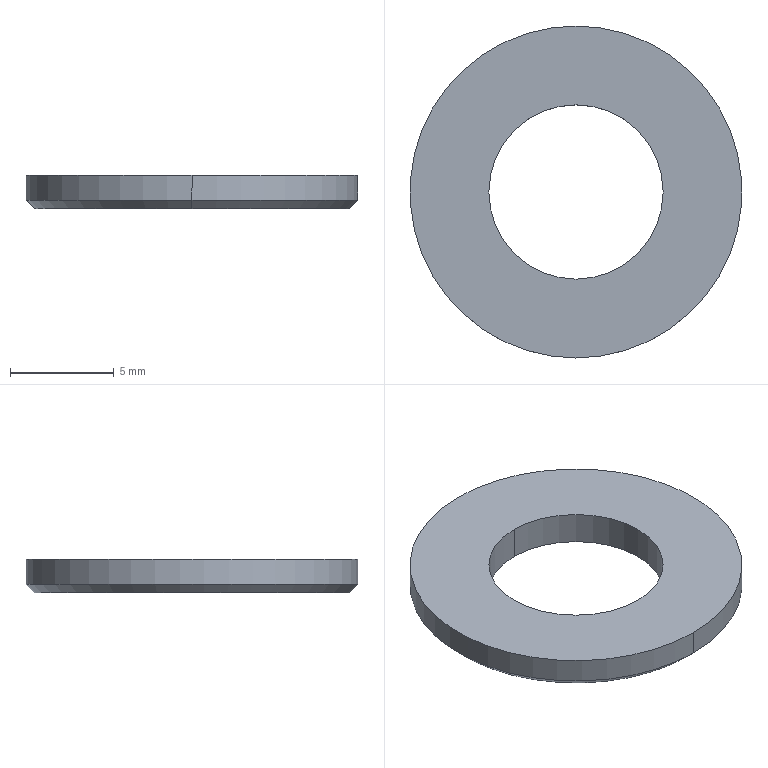Component | SolidWorks | GB_T97.2-1985FlatWasherChamferedTypeA8x1.6-10 | 1 solid | 8 faces | box 16 x 16 x 1.6 mm | volume 229 mm3 | cylinder 4 | cone 2 | plane 2 | commonest cylinder face diameters 16 x2 8.4 x2 | material Steel
build123d program:
from build123d import *


with BuildPart() as part:
    # Sketch1 → Base-Revolve (revolve)
    with BuildSketch(Plane.XY, mode=Mode.PRIVATE) as base_revolve_sk:
        Polygon((-7.6, 10.245), (-8, 9.845), (-8, 8.645), (-4.2, 8.645), (-4.2, 10.245), align=None)
    revolve(base_revolve_sk.sketch.rotate(Axis((0, 0, 0), (0, 1, 0)), 270), axis=Axis((0, 0, 0), (0, 1, 0)))


solid = part.part

# Placed as in the assembly
solid = solid.moved(Location((280, -19, -26.355), (-90, 0, 0)))
STEP:
#1=CARTESIAN_POINT('',(11.024,-1.063,-1.425));
#2=VERTEX_POINT('',#1);
#3=CARTESIAN_POINT('',(11.024,-0.4331,-1.425));
#4=VERTEX_POINT('',#3);
#5=CARTESIAN_POINT('',(11.024,-0.748,-1.425));
#6=DIRECTION('',(-0.,-0.,1.));
#7=DIRECTION('',(0.,-1.,-0.));
#8=AXIS2_PLACEMENT_3D('',#5,#6,#7);
#9=CIRCLE('',#8,0.315);
#10=EDGE_CURVE('',#2,#4,#9,.T.);
#11=ORIENTED_EDGE('',*,*,#10,.T.);
#12=CARTESIAN_POINT('',(11.024,-0.4331,-1.378));
#13=VERTEX_POINT('',#12);
#14=CARTESIAN_POINT('',(11.024,-0.4331,-1.038));
#15=DIRECTION('',(-0.,-0.,1.));
#16=VECTOR('',#15,39.37);
#17=LINE('',#14,#16);
#18=EDGE_CURVE('',#4,#13,#17,.T.);
#19=ORIENTED_EDGE('',*,*,#18,.T.);
#20=CARTESIAN_POINT('',(11.024,-1.063,-1.378));
#21=VERTEX_POINT('',#20);
#22=CARTESIAN_POINT('',(11.024,-0.748,-1.378));
#23=DIRECTION('',(-0.,-0.,1.));
#24=DIRECTION('',(0.,-1.,-0.));
#25=AXIS2_PLACEMENT_3D('',#22,#23,#24);
#26=CIRCLE('',#25,0.315);
#27=EDGE_CURVE('',#21,#13,#26,.T.);
#28=ORIENTED_EDGE('',*,*,#27,.F.);
#29=CARTESIAN_POINT('',(11.024,-1.063,-1.038));
#30=DIRECTION('',(-0.,-0.,1.));
#31=VECTOR('',#30,39.37);
#32=LINE('',#29,#31);
#33=EDGE_CURVE('',#2,#21,#32,.T.);
#34=ORIENTED_EDGE('',*,*,#33,.F.);
#35=EDGE_LOOP('',(#11,#19,#28,#34));
#36=FACE_OUTER_BOUND('',#35,.T.);
#37=CARTESIAN_POINT('',(11.024,-0.748,-1.038));
#38=DIRECTION('',(-0.,-0.,1.));
#39=DIRECTION('',(0.,-1.,-0.));
#40=AXIS2_PLACEMENT_3D('',#37,#38,#39);
#41=CYLINDRICAL_SURFACE('',#40,0.315);
#42=ADVANCED_FACE('',(#36),#41,.T.);
#43=CARTESIAN_POINT('',(11.024,-1.047,-1.441));
#44=VERTEX_POINT('',#43);
#45=CARTESIAN_POINT('',(11.024,-0.4488,-1.441));
#46=VERTEX_POINT('',#45);
#47=CARTESIAN_POINT('',(11.024,-0.748,-1.441));
#48=DIRECTION('',(-0.,-0.,1.));
#49=DIRECTION('',(0.,-1.,-0.));
#50=AXIS2_PLACEMENT_3D('',#47,#48,#49);
#51=CIRCLE('',#50,0.2992);
#52=EDGE_CURVE('',#44,#46,#51,.T.);
#53=ORIENTED_EDGE('',*,*,#52,.T.);
#54=CARTESIAN_POINT('',(11.024,-0.4488,-1.441));
#55=DIRECTION('',(-0.,0.7071,0.7071));
#56=VECTOR('',#55,39.37);
#57=LINE('',#54,#56);
#58=EDGE_CURVE('',#46,#4,#57,.T.);
#59=ORIENTED_EDGE('',*,*,#58,.T.);
#60=ORIENTED_EDGE('',*,*,#10,.F.);
#61=CARTESIAN_POINT('',(11.024,-1.047,-1.441));
#62=DIRECTION('',(-0.,-0.7071,0.7071));
#63=VECTOR('',#62,39.37);
#64=LINE('',#61,#63);
#65=EDGE_CURVE('',#44,#2,#64,.T.);
#66=ORIENTED_EDGE('',*,*,#65,.F.);
#67=EDGE_LOOP('',(#53,#59,#60,#66));
#68=FACE_OUTER_BOUND('',#67,.T.);
#69=CARTESIAN_POINT('',(11.024,-0.748,-1.441));
#70=DIRECTION('',(-0.,-0.,1.));
#71=DIRECTION('',(0.,-1.,-0.));
#72=AXIS2_PLACEMENT_3D('',#69,#70,#71);
#73=CONICAL_SURFACE('',#72,0.2992,0.7854);
#74=ADVANCED_FACE('',(#68),#73,.T.);
#75=CARTESIAN_POINT('',(11.024,-0.5827,-1.441));
#76=VERTEX_POINT('',#75);
#77=CARTESIAN_POINT('',(11.024,-0.9134,-1.441));
#78=VERTEX_POINT('',#77);
#79=CARTESIAN_POINT('',(11.024,-0.748,-1.441));
#80=DIRECTION('',(-0.,-0.,1.));
#81=DIRECTION('',(0.,-1.,-0.));
#82=AXIS2_PLACEMENT_3D('',#79,#80,#81);
#83=CIRCLE('',#82,0.1654);
#84=EDGE_CURVE('',#76,#78,#83,.T.);
#85=ORIENTED_EDGE('',*,*,#84,.F.);
#86=CARTESIAN_POINT('',(11.024,-0.5827,-1.378));
#87=VERTEX_POINT('',#86);
#88=CARTESIAN_POINT('',(11.024,-0.5827,-1.038));
#89=DIRECTION('',(-0.,-0.,1.));
#90=VECTOR('',#89,39.37);
#91=LINE('',#88,#90);
#92=EDGE_CURVE('',#76,#87,#91,.T.);
#93=ORIENTED_EDGE('',*,*,#92,.T.);
#94=CARTESIAN_POINT('',(11.024,-0.9134,-1.378));
#95=VERTEX_POINT('',#94);
#96=CARTESIAN_POINT('',(11.024,-0.748,-1.378));
#97=DIRECTION('',(-0.,-0.,1.));
#98=DIRECTION('',(0.,-1.,-0.));
#99=AXIS2_PLACEMENT_3D('',#96,#97,#98);
#100=CIRCLE('',#99,0.1654);
#101=EDGE_CURVE('',#87,#95,#100,.T.);
#102=ORIENTED_EDGE('',*,*,#101,.T.);
#103=CARTESIAN_POINT('',(11.024,-0.9134,-1.038));
#104=DIRECTION('',(-0.,-0.,1.));
#105=VECTOR('',#104,39.37);
#106=LINE('',#103,#105);
#107=EDGE_CURVE('',#78,#95,#106,.T.);
#108=ORIENTED_EDGE('',*,*,#107,.F.);
#109=EDGE_LOOP('',(#85,#93,#102,#108));
#110=FACE_OUTER_BOUND('',#109,.T.);
#111=CARTESIAN_POINT('',(11.024,-0.748,-1.038));
#112=DIRECTION('',(-0.,-0.,1.));
#113=DIRECTION('',(0.,-1.,-0.));
#114=AXIS2_PLACEMENT_3D('',#111,#112,#113);
#115=CYLINDRICAL_SURFACE('',#114,0.1654);
#116=ADVANCED_FACE('',(#110),#115,.F.);
#117=ORIENTED_EDGE('',*,*,#92,.F.);
#118=CARTESIAN_POINT('',(11.024,-0.748,-1.441));
#119=DIRECTION('',(-0.,-0.,1.));
#120=DIRECTION('',(0.,-1.,-0.));
#121=AXIS2_PLACEMENT_3D('',#118,#119,#120);
#122=CIRCLE('',#121,0.1654);
#123=EDGE_CURVE('',#78,#76,#122,.T.);
#124=ORIENTED_EDGE('',*,*,#123,.F.);
#125=ORIENTED_EDGE('',*,*,#107,.T.);
#126=CARTESIAN_POINT('',(11.024,-0.748,-1.378));
#127=DIRECTION('',(-0.,-0.,1.));
#128=DIRECTION('',(0.,-1.,-0.));
#129=AXIS2_PLACEMENT_3D('',#126,#127,#128);
#130=CIRCLE('',#129,0.1654);
#131=EDGE_CURVE('',#95,#87,#130,.T.);
#132=ORIENTED_EDGE('',*,*,#131,.T.);
#133=EDGE_LOOP('',(#117,#124,#125,#132));
#134=FACE_OUTER_BOUND('',#133,.T.);
#135=CARTESIAN_POINT('',(11.024,-0.748,-1.038));
#136=DIRECTION('',(-0.,-0.,1.));
#137=DIRECTION('',(0.,-1.,-0.));
#138=AXIS2_PLACEMENT_3D('',#135,#136,#137);
#139=CYLINDRICAL_SURFACE('',#138,0.1654);
#140=ADVANCED_FACE('',(#134),#139,.F.);
#141=ORIENTED_EDGE('',*,*,#52,.F.);
#142=CARTESIAN_POINT('',(11.024,-0.748,-1.441));
#143=DIRECTION('',(-0.,-0.,1.));
#144=DIRECTION('',(0.,-1.,-0.));
#145=AXIS2_PLACEMENT_3D('',#142,#143,#144);
#146=CIRCLE('',#145,0.2992);
#147=EDGE_CURVE('',#46,#44,#146,.T.);
#148=ORIENTED_EDGE('',*,*,#147,.F.);
#149=EDGE_LOOP('',(#141,#148));
#150=FACE_OUTER_BOUND('',#149,.T.);
#151=ORIENTED_EDGE('',*,*,#123,.T.);
#152=ORIENTED_EDGE('',*,*,#84,.T.);
#153=EDGE_LOOP('',(#151,#152));
#154=FACE_BOUND('',#153,.T.);
#155=CARTESIAN_POINT('',(10.858,-0.748,-1.441));
#156=DIRECTION('',(-0.,-0.,1.));
#157=DIRECTION('',(0.,-1.,-0.));
#158=AXIS2_PLACEMENT_3D('',#155,#156,#157);
#159=PLANE('',#158);
#160=ADVANCED_FACE('',(#150,#154),#159,.F.);
#161=ORIENTED_EDGE('',*,*,#58,.F.);
#162=ORIENTED_EDGE('',*,*,#147,.T.);
#163=ORIENTED_EDGE('',*,*,#65,.T.);
#164=CARTESIAN_POINT('',(11.024,-0.748,-1.425));
#165=DIRECTION('',(-0.,-0.,1.));
#166=DIRECTION('',(0.,-1.,-0.));
#167=AXIS2_PLACEMENT_3D('',#164,#165,#166);
#168=CIRCLE('',#167,0.315);
#169=EDGE_CURVE('',#4,#2,#168,.T.);
#170=ORIENTED_EDGE('',*,*,#169,.F.);
#171=EDGE_LOOP('',(#161,#162,#163,#170));
#172=FACE_OUTER_BOUND('',#171,.T.);
#173=CARTESIAN_POINT('',(11.024,-0.748,-1.441));
#174=DIRECTION('',(-0.,-0.,1.));
#175=DIRECTION('',(0.,-1.,-0.));
#176=AXIS2_PLACEMENT_3D('',#173,#174,#175);
#177=CONICAL_SURFACE('',#176,0.2992,0.7854);
#178=ADVANCED_FACE('',(#172),#177,.T.);
#179=ORIENTED_EDGE('',*,*,#18,.F.);
#180=ORIENTED_EDGE('',*,*,#169,.T.);
#181=ORIENTED_EDGE('',*,*,#33,.T.);
#182=CARTESIAN_POINT('',(11.024,-0.748,-1.378));
#183=DIRECTION('',(-0.,-0.,1.));
#184=DIRECTION('',(0.,-1.,-0.));
#185=AXIS2_PLACEMENT_3D('',#182,#183,#184);
#186=CIRCLE('',#185,0.315);
#187=EDGE_CURVE('',#13,#21,#186,.T.);
#188=ORIENTED_EDGE('',*,*,#187,.F.);
#189=EDGE_LOOP('',(#179,#180,#181,#188));
#190=FACE_OUTER_BOUND('',#189,.T.);
#191=CARTESIAN_POINT('',(11.024,-0.748,-1.038));
#192=DIRECTION('',(-0.,-0.,1.));
#193=DIRECTION('',(0.,-1.,-0.));
#194=AXIS2_PLACEMENT_3D('',#191,#192,#193);
#195=CYLINDRICAL_SURFACE('',#194,0.315);
#196=ADVANCED_FACE('',(#190),#195,.T.);
#197=ORIENTED_EDGE('',*,*,#131,.F.);
#198=ORIENTED_EDGE('',*,*,#101,.F.);
#199=EDGE_LOOP('',(#197,#198));
#200=FACE_BOUND('',#199,.T.);
#201=ORIENTED_EDGE('',*,*,#27,.T.);
#202=ORIENTED_EDGE('',*,*,#187,.T.);
#203=EDGE_LOOP('',(#201,#202));
#204=FACE_OUTER_BOUND('',#203,.T.);
#205=CARTESIAN_POINT('',(10.858,-0.748,-1.378));
#206=DIRECTION('',(0.,0.,-1.));
#207=DIRECTION('',(-0.,1.,0.));
#208=AXIS2_PLACEMENT_3D('',#205,#206,#207);
#209=PLANE('',#208);
#210=ADVANCED_FACE('',(#200,#204),#209,.F.);
#211=CLOSED_SHELL('',(#42,#74,#116,#140,#160,#178,#196,#210));
#212=MANIFOLD_SOLID_BREP('',#211);
#213=CARTESIAN_POINT('',(0.,0.,0.));
#214=DIRECTION('',(0.,0.,1.));
#215=DIRECTION('',(1.,0.,0.));
#216=AXIS2_PLACEMENT_3D('',#213,#214,#215);
#217=(LENGTH_UNIT()NAMED_UNIT(*)SI_UNIT($,.METRE.));
#218=LENGTH_MEASURE_WITH_UNIT(LENGTH_MEASURE(0.0254),#217);
#219=DIMENSIONAL_EXPONENTS(1.,0.,0.,0.,0.,0.,0.);
#220=(CONVERSION_BASED_UNIT('',#218)LENGTH_UNIT()NAMED_UNIT(#219));
#221=UNCERTAINTY_MEASURE_WITH_UNIT(LENGTH_MEASURE(0.00001),#220,'','');
#222=(NAMED_UNIT(*)PLANE_ANGLE_UNIT()SI_UNIT($,.RADIAN.));
#223=(NAMED_UNIT(*)SI_UNIT($,.STERADIAN.)SOLID_ANGLE_UNIT());
#224=(GEOMETRIC_REPRESENTATION_CONTEXT(3)GLOBAL_UNCERTAINTY_ASSIGNED_CONTEXT((#221))GLOBAL_UNIT_ASSIGNED_CONTEXT((#220,#222,#223))REPRESENTATION_CONTEXT('',''));
#225=ADVANCED_BREP_SHAPE_REPRESENTATION('',(#212,#216),#224);
#226=COLOUR_RGB('',0.7922,0.8196,0.9333);
#227=FILL_AREA_STYLE_COLOUR('',#226);
#228=FILL_AREA_STYLE('',(#227));
#229=SURFACE_STYLE_FILL_AREA(#228);
#230=SURFACE_SIDE_STYLE('',(#229));
#231=SURFACE_STYLE_USAGE(.BOTH.,#230);
#232=PRESENTATION_STYLE_ASSIGNMENT((#231));
#233=STYLED_ITEM('',(#232),#212);
#234=(LENGTH_UNIT()NAMED_UNIT(*)SI_UNIT($,.METRE.));
#235=LENGTH_MEASURE_WITH_UNIT(LENGTH_MEASURE(0.0254),#234);
#236=DIMENSIONAL_EXPONENTS(1.,0.,0.,0.,0.,0.,0.);
#237=(CONVERSION_BASED_UNIT('',#235)LENGTH_UNIT()NAMED_UNIT(#236));
#238=UNCERTAINTY_MEASURE_WITH_UNIT(LENGTH_MEASURE(0.00001),#237,'','');
#239=(NAMED_UNIT(*)PLANE_ANGLE_UNIT()SI_UNIT($,.RADIAN.));
#240=(NAMED_UNIT(*)SI_UNIT($,.STERADIAN.)SOLID_ANGLE_UNIT());
#241=(GEOMETRIC_REPRESENTATION_CONTEXT(3)GLOBAL_UNCERTAINTY_ASSIGNED_CONTEXT((#238))GLOBAL_UNIT_ASSIGNED_CONTEXT((#237,#239,#240))REPRESENTATION_CONTEXT('',''));
#242=MECHANICAL_DESIGN_GEOMETRIC_PRESENTATION_REPRESENTATION('',(#233),#241);
#243=PRESENTATION_LAYER_ASSIGNMENT('','',(#233));